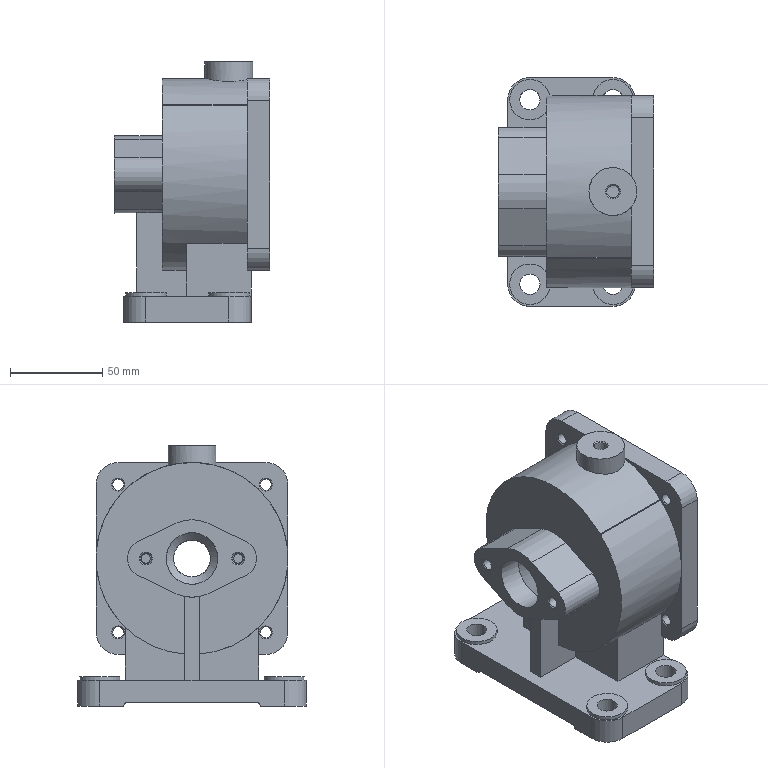Component | NX | PUMP_BODY | 1 solid | 100 faces | volume 423481 mm3 | plane 46 | cylinder 40 | cone 13 | spline 1 | commonest cylinder face diameters 24 x8 6 x6 22 x4 11 x4 104 x3 20 x3 5 x3 42 x2